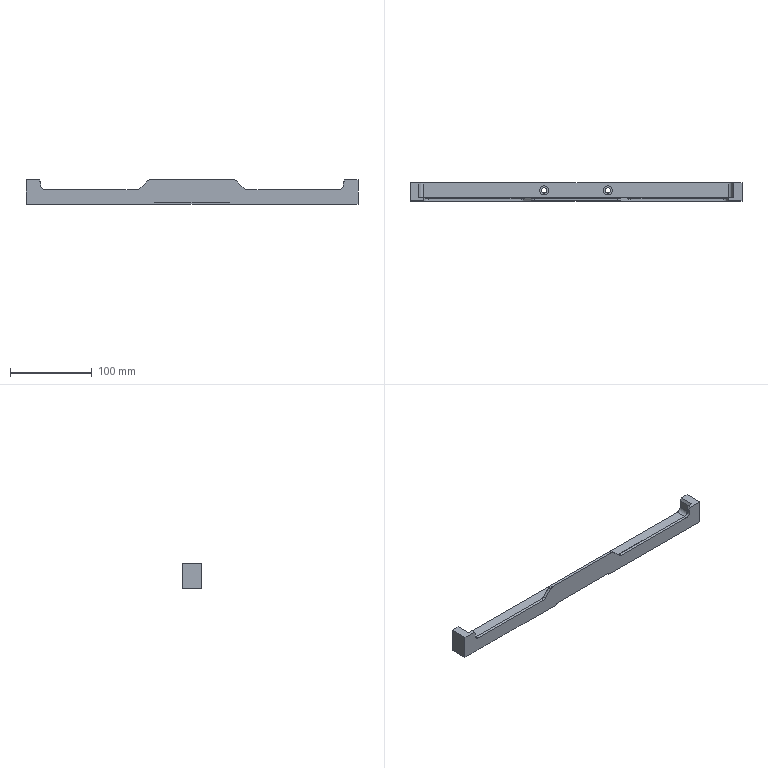Component | SolidWorks | MGPM25-20Z-A93LAssembly-1_30-33A-1 | 1 solid | 59 faces | box 405 x 22 x 30 mm | volume 126911 mm3 | plane 35 | cylinder 18 | cone 6 | commonest cylinder face diameters 10 x8 6.6 x4 11 x4 2 x2
build123d program:
from build123d import *
from OCP.BRepFilletAPI import BRepFilletAPI_MakeChamfer

# Parameters (mm, degrees)
SKETCH1_W                                            = 18
SKETCH1_H                                            = 22
EXTRUDE1_DEPTH                                       = 202.5
CUT_EXTRUDE1_DEPTH                                   = 18
COUNTERBORE_FOR_M6_HEXAGON_SOCKET_HEAD_C_D           = 6.6
COUNTERBORE_FOR_M6_HEXAGON_SOCKET_HEAD_C_CBORE_D     = 11
COUNTERBORE_FOR_M6_HEXAGON_SOCKET_HEAD_C_CBORE_DEPTH = 6.5
EXTRUDE6_DEPTH                                       = 4
CUT_EXTRUDE6_DEPTH                                   = 2
EXTRUDE7_DEPTH                                       = 12
FILLET2_R                                            = 5
CHAMFER9_SIZE                                        = 0.5
CHAMFER10_SIZE                                       = 2
CHAMFER10_SIZE2                                      = 3.464


with BuildPart() as part:
    # Sketch1 → Extrude1 (new, symmetric)
    with BuildSketch(Plane.XY):
        with Locations((-9, 11)):
            Rectangle(SKETCH1_W, SKETCH1_H)
    extrude(amount=EXTRUDE1_DEPTH, both=True)

    # Sketch28 → Cut-Extrude1 (cut)
    with BuildSketch(Plane(origin=(0, 22, 0), x_dir=(1, 0, 0), z_dir=(0, 1, 0))):
        with BuildLine():
            Line((-18, 190.5), (-17, 190.5))
            ThreePointArc((-17, 190.5), (-13.464, 189.036), (-12, 185.5))
            Line((-12, 185.5), (-12, -185.5))
            ThreePointArc((-12, -185.5), (-13.464, -189.036), (-17, -190.5))
            Line((-17, -190.5), (-18, -190.5))
            Line((-18, -190.5), (-18, 190.5))
        make_face()
    extrude(amount=-CUT_EXTRUDE1_DEPTH, mode=Mode.SUBTRACT)

    # Counterbore for M6 Hexagon Socket Head C (through all)
    with Locations(Plane(origin=(-12, 8.28, -125.712), x_dir=(0, 0, 1), z_dir=(-1, 0, 0))):
        with Locations((86.712, 4.72), (164.712, 4.72)):
            CounterBoreHole(COUNTERBORE_FOR_M6_HEXAGON_SOCKET_HEAD_C_D / 2, COUNTERBORE_FOR_M6_HEXAGON_SOCKET_HEAD_C_CBORE_D / 2, COUNTERBORE_FOR_M6_HEXAGON_SOCKET_HEAD_C_CBORE_DEPTH)

    # Sketch31 → Extrude6 (add)
    with BuildSketch(Plane(origin=(0, 4, 0), x_dir=(1, 0, 0), z_dir=(0, 1, 0))):
        Polygon((-18, -65), (-30, -53), (-30, 53), (-18, 65), align=None)
    extrude(amount=-EXTRUDE6_DEPTH)

    # Sketch34 → Cut-Extrude6 (cut)
    with BuildSketch(Plane(origin=(0, 0, 0), x_dir=(0, 0, -1), z_dir=(1, 0, 0))):
        with BuildLine():
            Line((-45.5, -15), (45.5, -15))
            Line((45.5, -15), (45.5, 18))
            ThreePointArc((45.5, 18), (45.207, 18.707), (44.5, 19))
            Line((44.5, 19), (-44.5, 19))
            ThreePointArc((-44.5, 19), (-45.207, 18.707), (-45.5, 18))
            Line((-45.5, 18), (-45.5, -15))
        make_face()
    extrude(amount=-CUT_EXTRUDE6_DEPTH, mode=Mode.SUBTRACT)

    # Sketch35 → Extrude7 (add)
    with BuildSketch(Plane.ZY.offset(18)):
        Polygon((-202.5, 22), (-190.5, 22), (-190.5, 4), (-184.5, 4), (-184.5, 0), (-202.5, 0), align=None)
        Polygon((184.5, 4), (184.5, 0), (202.5, 0), (202.5, 22), (190.5, 22), (190.5, 4), align=None)
    extrude(amount=EXTRUDE7_DEPTH)

    # Fillet2
    fillet2_edges = [part.edges().sort_by_distance(p)[0] for p in [
        (-18, 2, 65),
        (-30, 2, 53),
        (-30, 2, -53),
        (-18, 2, -65),
        (-18, 2, 184.5),
        (-18, 2, -184.5),
    ]]
    fillet(fillet2_edges, radius=FILLET2_R)

    # Chamfer9
    chamfer9_edges = [part.edges().sort_by_distance(p)[0] for p in [
        (-26.5, 4, 184.5),
        (-18, 4, 123.286),
        (-18, 4, -123.286),
        (-24, 4, 59),
        (-30, 4, 0),
        (-24, 4, -59),
        (-29.619, 4, -52.842),
        (-29.619, 4, 52.842),
        (-19.464, 4, 183.036),
        (-19.464, 4, -183.036),
        (-18.381, 4, 65.158),
        (-18.381, 4, -65.158),
        (-26.5, 4, -184.5),
    ]]
    chamfer(chamfer9_edges, length=CHAMFER9_SIZE)

    # Chamfer10: one chamfer whose edges measure the first distance from different faces: ONE call of the kernel's chamfer builder (chamfer() names one face for all edges)
    chamfer10_edges_1 = [part.edges().sort_by_distance(p)[0] for p in [
        (-30, 13, -190.5),
        (-30, 1.75, -184.5),
    ]]
    chamfer10_side_1 = [part.faces().sort_by_distance(p)[0] for p in [
        (-30, 10.253, -195.755),
    ]]
    chamfer10_edges_2 = [part.edges().sort_by_distance(p)[0] for p in [
        (-30, 13, 190.5),
        (-30, 1.75, 184.5),
    ]]
    chamfer10_side_2 = [part.faces().sort_by_distance(p)[0] for p in [
        (-30, 10.253, 195.755),
    ]]
    chamfer10 = BRepFilletAPI_MakeChamfer(part.part.solid().wrapped)
    for e in chamfer10_edges_1:
        chamfer10.Add(CHAMFER10_SIZE, CHAMFER10_SIZE2, e.wrapped, chamfer10_side_1[0].wrapped)  # the first distance lies on this face
    for e in chamfer10_edges_2:
        chamfer10.Add(CHAMFER10_SIZE, CHAMFER10_SIZE2, e.wrapped, chamfer10_side_2[0].wrapped)  # the first distance lies on this face
    add(Compound.cast(chamfer10.Shape()), mode=Mode.REPLACE)


solid = part.part

# Placed as in the assembly
solid = solid.moved(Location((-649.208, -2.092, 148.188), (0, 90, 0)))